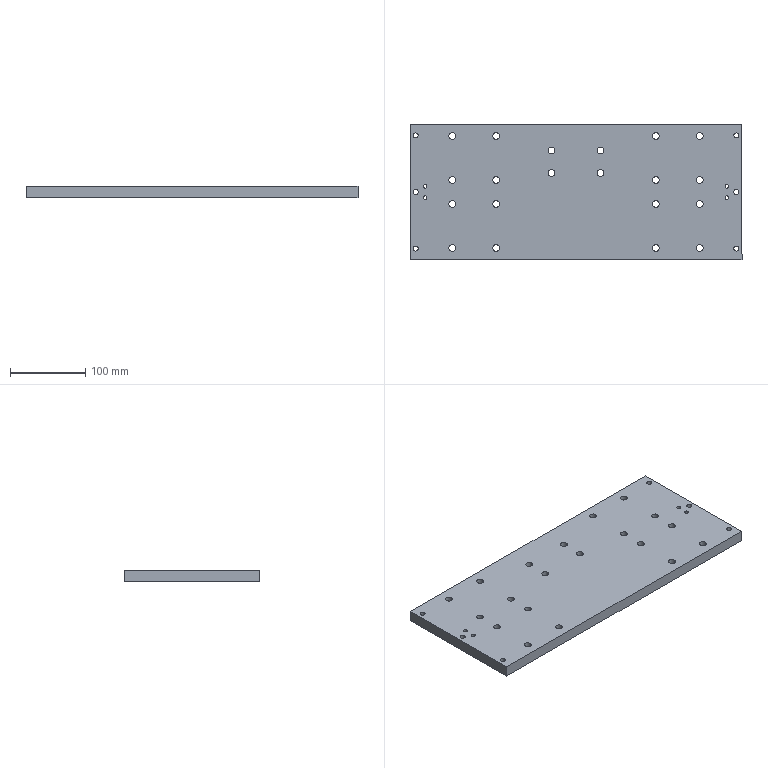Component | SolidWorks | 30-20A-1 | 1 solid | 84 faces | box 440 x 180 x 15 mm | volume 1162468 mm3 | cylinder 72 | plane 12 | commonest cylinder face diameters 9 x40 11 x12 6.6 x12 5 x8
build123d program:
from build123d import *

# Parameters (mm, degrees)
SKETCH1_W                                         = 440
SKETCH1_H                                         = 180
EXTRUDE1_DEPTH                                    = 15
SKETCH5_R                                         = 4.5
CUT_EXTRUDE1_DEPTH                                = 15
LINEAR_PATTERN3_COUNT                             = 2
LINEAR_PATTERN3_PITCH                             = 58
LINEAR_PATTERN3_COUNT_DIR2                        = 2
LINEAR_PATTERN3_PITCH_DIR2                        = 58
MIRROR1_COPY_1_SKETCH_R                           = 4.5
MIRROR1_COPY_1_DEPTH                              = 15
MIRROR1_COPY_2_SKETCH_R                           = 4.5
MIRROR1_COPY_2_DEPTH                              = 15
MIRROR1_COPY_3_SKETCH_R                           = 4.5
MIRROR1_COPY_3_DEPTH                              = 15
MIRROR2_COPY_1_SKETCH_R                           = 4.5
MIRROR2_COPY_1_DEPTH                              = 15
MIRROR2_COPY_2_SKETCH_R                           = 4.5
MIRROR2_COPY_2_DEPTH                              = 15
MIRROR2_COPY_3_SKETCH_R                           = 4.5
MIRROR2_COPY_3_DEPTH                              = 15
MIRROR2_COPY_4_SKETCH_R                           = 4.5
MIRROR2_COPY_4_DEPTH                              = 15
MIRROR2_COPY_5_SKETCH_R                           = 4.5
MIRROR2_COPY_5_DEPTH                              = 15
MIRROR2_COPY_6_SKETCH_R                           = 4.5
MIRROR2_COPY_6_DEPTH                              = 15
MIRROR2_COPY_7_SKETCH_R                           = 4.5
MIRROR2_COPY_7_DEPTH                              = 15
M6_TAPPED_HOLE1_D                                 = 5
M6_SOCKET_HEAD_CAP_SCREW_COUNTERBORE2_D           = 6.6
M6_SOCKET_HEAD_CAP_SCREW_COUNTERBORE2_CBORE_D     = 11
M6_SOCKET_HEAD_CAP_SCREW_COUNTERBORE2_CBORE_DEPTH = 6
F_9_0_9_DIAMETER_HOLE1_D                          = 9


with BuildPart() as part:
    # Sketch1 → Extrude1 (new body)
    with BuildSketch(Plane.XY):
        Rectangle(SKETCH1_W, SKETCH1_H)
    extrude(amount=EXTRUDE1_DEPTH)

    # Sketch5 → Cut-Extrude1 (cut)
    with BuildSketch(Plane.XY.offset(15)):
        with Locations((106, 74)):
            Circle(SKETCH5_R)
    cut_extrude1 = extrude(amount=-CUT_EXTRUDE1_DEPTH, mode=Mode.SUBTRACT)

    # Linear Pattern3: Cut-Extrude1 2 × 2
    with Locations(*[(i * LINEAR_PATTERN3_PITCH, -j * LINEAR_PATTERN3_PITCH_DIR2, 0) for i in range(LINEAR_PATTERN3_COUNT) for j in range(LINEAR_PATTERN3_COUNT_DIR2) if (i, j) != (0, 0)]):
        add(cut_extrude1, mode=Mode.SUBTRACT)

    # Mirror1: Cut-Extrude1 across plane
    add(cut_extrude1.mirror(Plane(origin=(0, 0, 0), x_dir=(0, 0, 1), z_dir=(1, 0, 0))), mode=Mode.SUBTRACT)

    # Mirror1 copy 1 sketch → Mirror1 copy 1 (cut)
    with BuildSketch(Plane(origin=(0, -58, 15), x_dir=(-1, 0, 0), z_dir=(0, 0, 1))):
        with Locations((106, -74)):
            Circle(MIRROR1_COPY_1_SKETCH_R)
    extrude(amount=-MIRROR1_COPY_1_DEPTH, mode=Mode.SUBTRACT)

    # Mirror1 copy 2 sketch → Mirror1 copy 2 (cut)
    with BuildSketch(Plane(origin=(-58, 0, 15), x_dir=(-1, 0, 0), z_dir=(0, 0, 1))):
        with Locations((106, -74)):
            Circle(MIRROR1_COPY_2_SKETCH_R)
    extrude(amount=-MIRROR1_COPY_2_DEPTH, mode=Mode.SUBTRACT)

    # Mirror1 copy 3 sketch → Mirror1 copy 3 (cut)
    with BuildSketch(Plane(origin=(-58, -58, 15), x_dir=(-1, 0, 0), z_dir=(0, 0, 1))):
        with Locations((106, -74)):
            Circle(MIRROR1_COPY_3_SKETCH_R)
    extrude(amount=-MIRROR1_COPY_3_DEPTH, mode=Mode.SUBTRACT)

    # Mirror2: Cut-Extrude1 across plane
    add(cut_extrude1.mirror(Plane.ZX), mode=Mode.SUBTRACT)

    # Mirror2 copy 1 sketch → Mirror2 copy 1 (cut)
    with BuildSketch(Plane(origin=(0, 58, 15), x_dir=(1, 0, 0), z_dir=(0, 0, 1))):
        with Locations((106, -74)):
            Circle(MIRROR2_COPY_1_SKETCH_R)
    extrude(amount=-MIRROR2_COPY_1_DEPTH, mode=Mode.SUBTRACT)

    # Mirror2 copy 2 sketch → Mirror2 copy 2 (cut)
    with BuildSketch(Plane(origin=(58, 0, 15), x_dir=(1, 0, 0), z_dir=(0, 0, 1))):
        with Locations((106, -74)):
            Circle(MIRROR2_COPY_2_SKETCH_R)
    extrude(amount=-MIRROR2_COPY_2_DEPTH, mode=Mode.SUBTRACT)

    # Mirror2 copy 3 sketch → Mirror2 copy 3 (cut)
    with BuildSketch(Plane(origin=(58, 58, 15), x_dir=(1, 0, 0), z_dir=(0, 0, 1))):
        with Locations((106, -74)):
            Circle(MIRROR2_COPY_3_SKETCH_R)
    extrude(amount=-MIRROR2_COPY_3_DEPTH, mode=Mode.SUBTRACT)

    # Mirror2 copy 4 sketch → Mirror2 copy 4 (cut)
    with BuildSketch(Plane(origin=(0, 0, 15), x_dir=(-1, 0, 0), z_dir=(0, 0, 1))):
        with Locations((106, 74)):
            Circle(MIRROR2_COPY_4_SKETCH_R)
    extrude(amount=-MIRROR2_COPY_4_DEPTH, mode=Mode.SUBTRACT)

    # Mirror2 copy 5 sketch → Mirror2 copy 5 (cut)
    with BuildSketch(Plane(origin=(0, 58, 15), x_dir=(-1, 0, 0), z_dir=(0, 0, 1))):
        with Locations((106, 74)):
            Circle(MIRROR2_COPY_5_SKETCH_R)
    extrude(amount=-MIRROR2_COPY_5_DEPTH, mode=Mode.SUBTRACT)

    # Mirror2 copy 6 sketch → Mirror2 copy 6 (cut)
    with BuildSketch(Plane(origin=(-58, 0, 15), x_dir=(-1, 0, 0), z_dir=(0, 0, 1))):
        with Locations((106, 74)):
            Circle(MIRROR2_COPY_6_SKETCH_R)
    extrude(amount=-MIRROR2_COPY_6_DEPTH, mode=Mode.SUBTRACT)

    # Mirror2 copy 7 sketch → Mirror2 copy 7 (cut)
    with BuildSketch(Plane(origin=(-58, 58, 15), x_dir=(-1, 0, 0), z_dir=(0, 0, 1))):
        with Locations((106, 74)):
            Circle(MIRROR2_COPY_7_SKETCH_R)
    extrude(amount=-MIRROR2_COPY_7_DEPTH, mode=Mode.SUBTRACT)

    # M6 Tapped Hole1 (through all)
    with Locations(Plane.XY.offset(15)):
        with Locations((-200, 7.5), (-200, -7.5), (200, -7.5), (200, 7.5)):
            Hole(M6_TAPPED_HOLE1_D / 2)

    # M6 Socket Head Cap Screw Counterbore2 (through all)
    with Locations(Plane.XY.offset(15)):
        with Locations((-212.5, -75), (-212.5, 0), (-212.5, 75), (212.5, 75), (212.5, 0), (212.5, -75)):
            CounterBoreHole(M6_SOCKET_HEAD_CAP_SCREW_COUNTERBORE2_D / 2, M6_SOCKET_HEAD_CAP_SCREW_COUNTERBORE2_CBORE_D / 2, M6_SOCKET_HEAD_CAP_SCREW_COUNTERBORE2_CBORE_DEPTH)

    # 9.0 _9_ Diameter Hole1 (through all)
    with Locations(Plane.XY.offset(15)):
        with Locations((32.5, -25), (32.5, -55), (-32.5, -55), (-32.5, -25)):
            Hole(F_9_0_9_DIAMETER_HOLE1_D / 2)


solid = part.part

# Placed as in the assembly
solid = solid.moved(Location((-649.208, -77.092, 39.188), (180, 0, 0)))